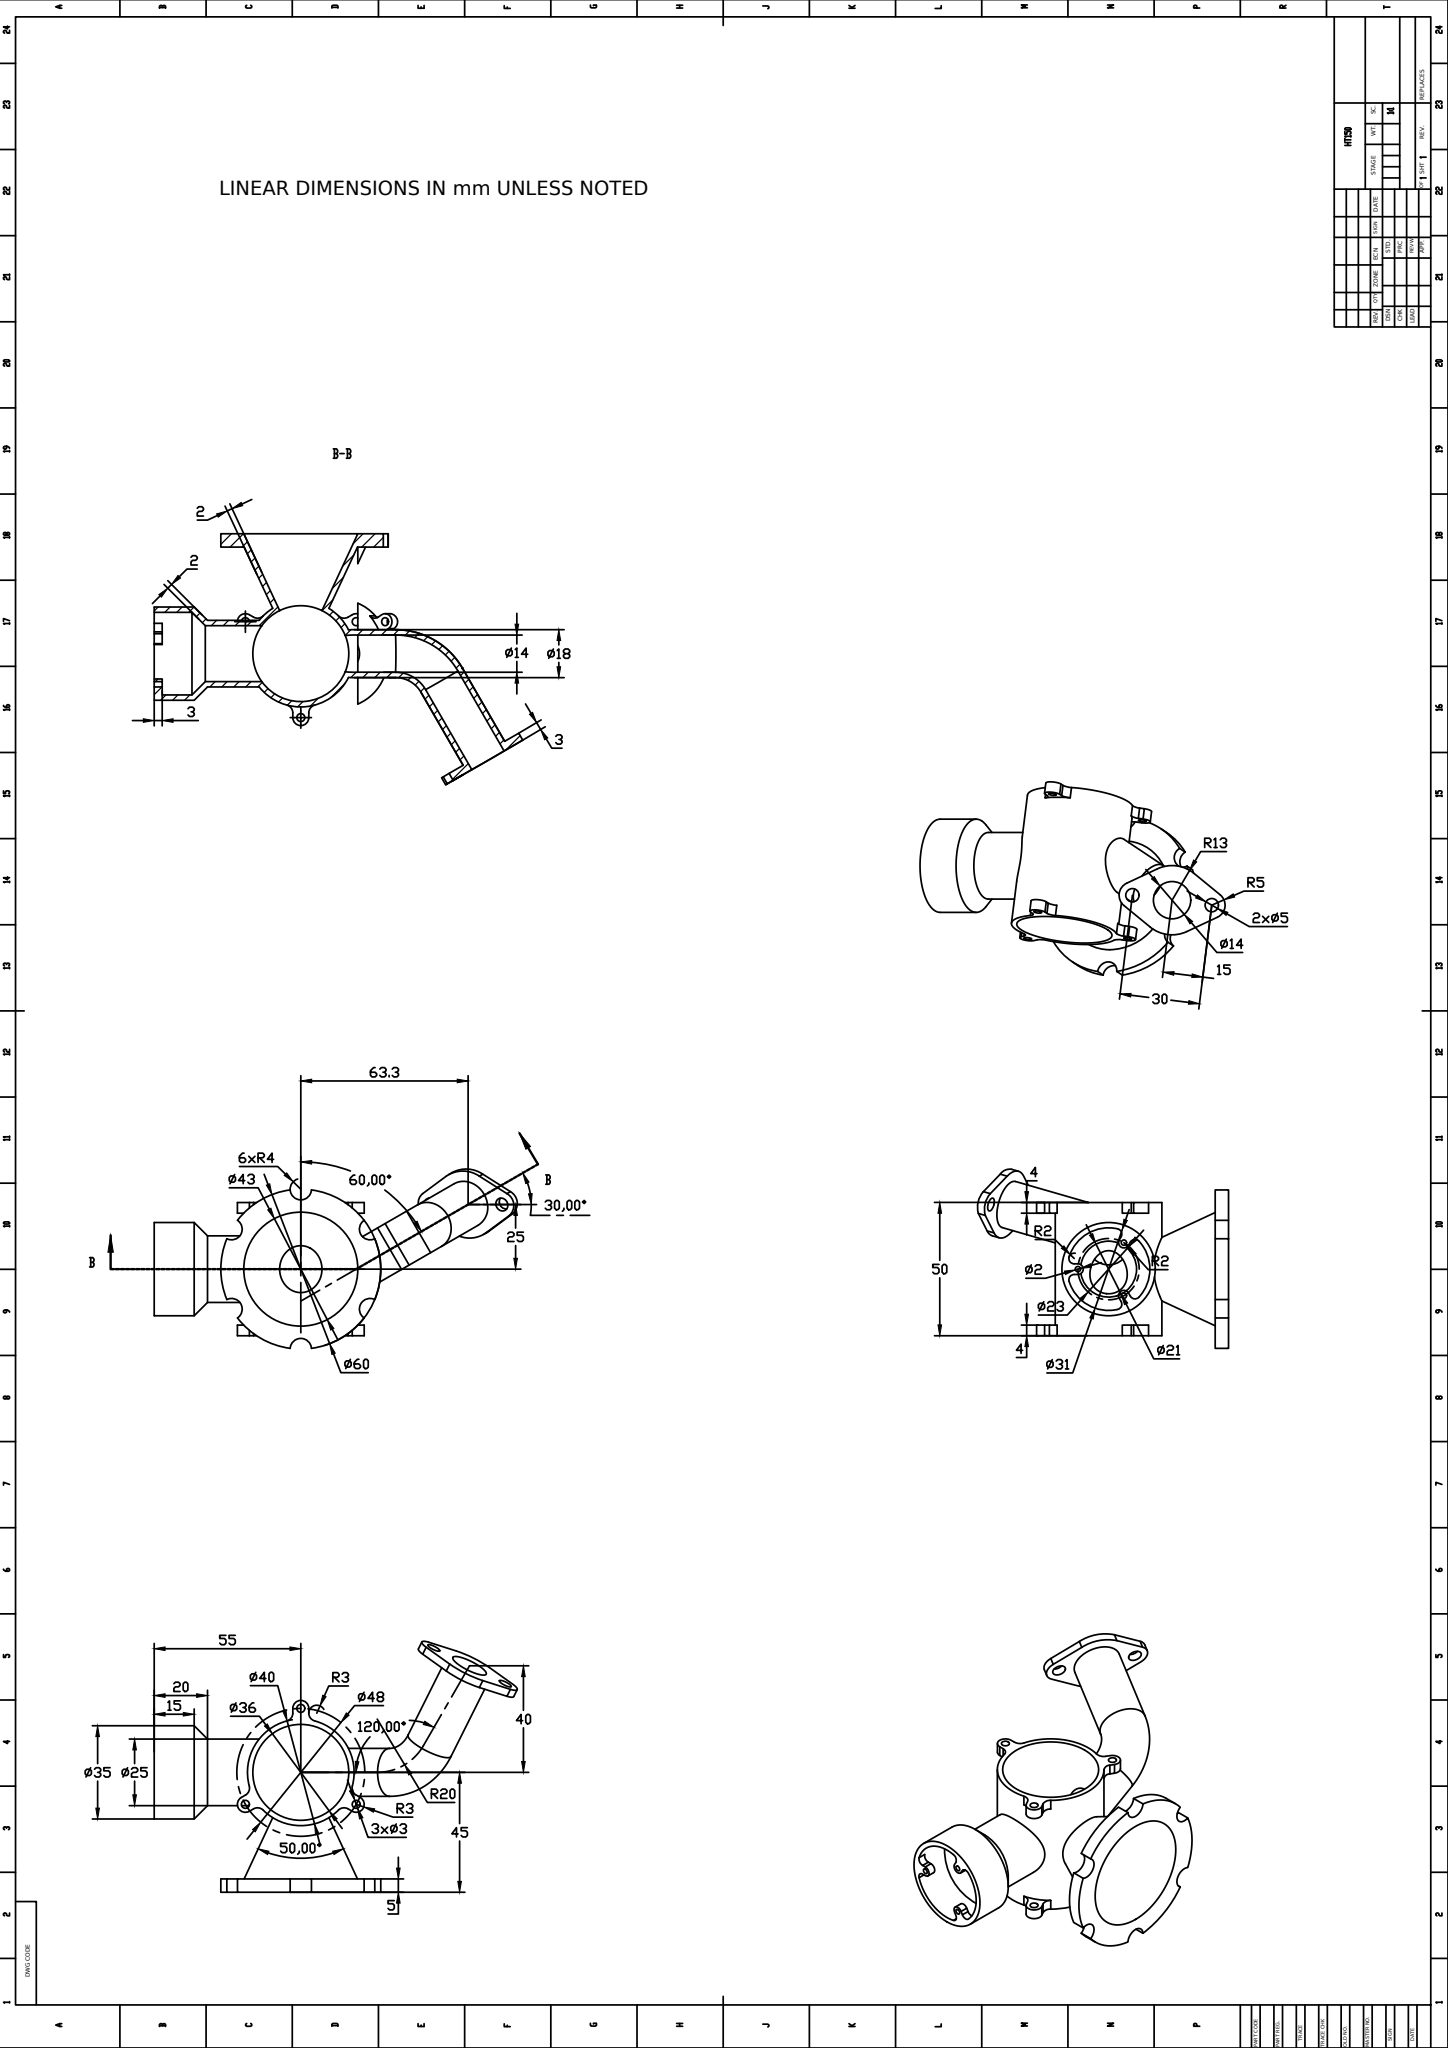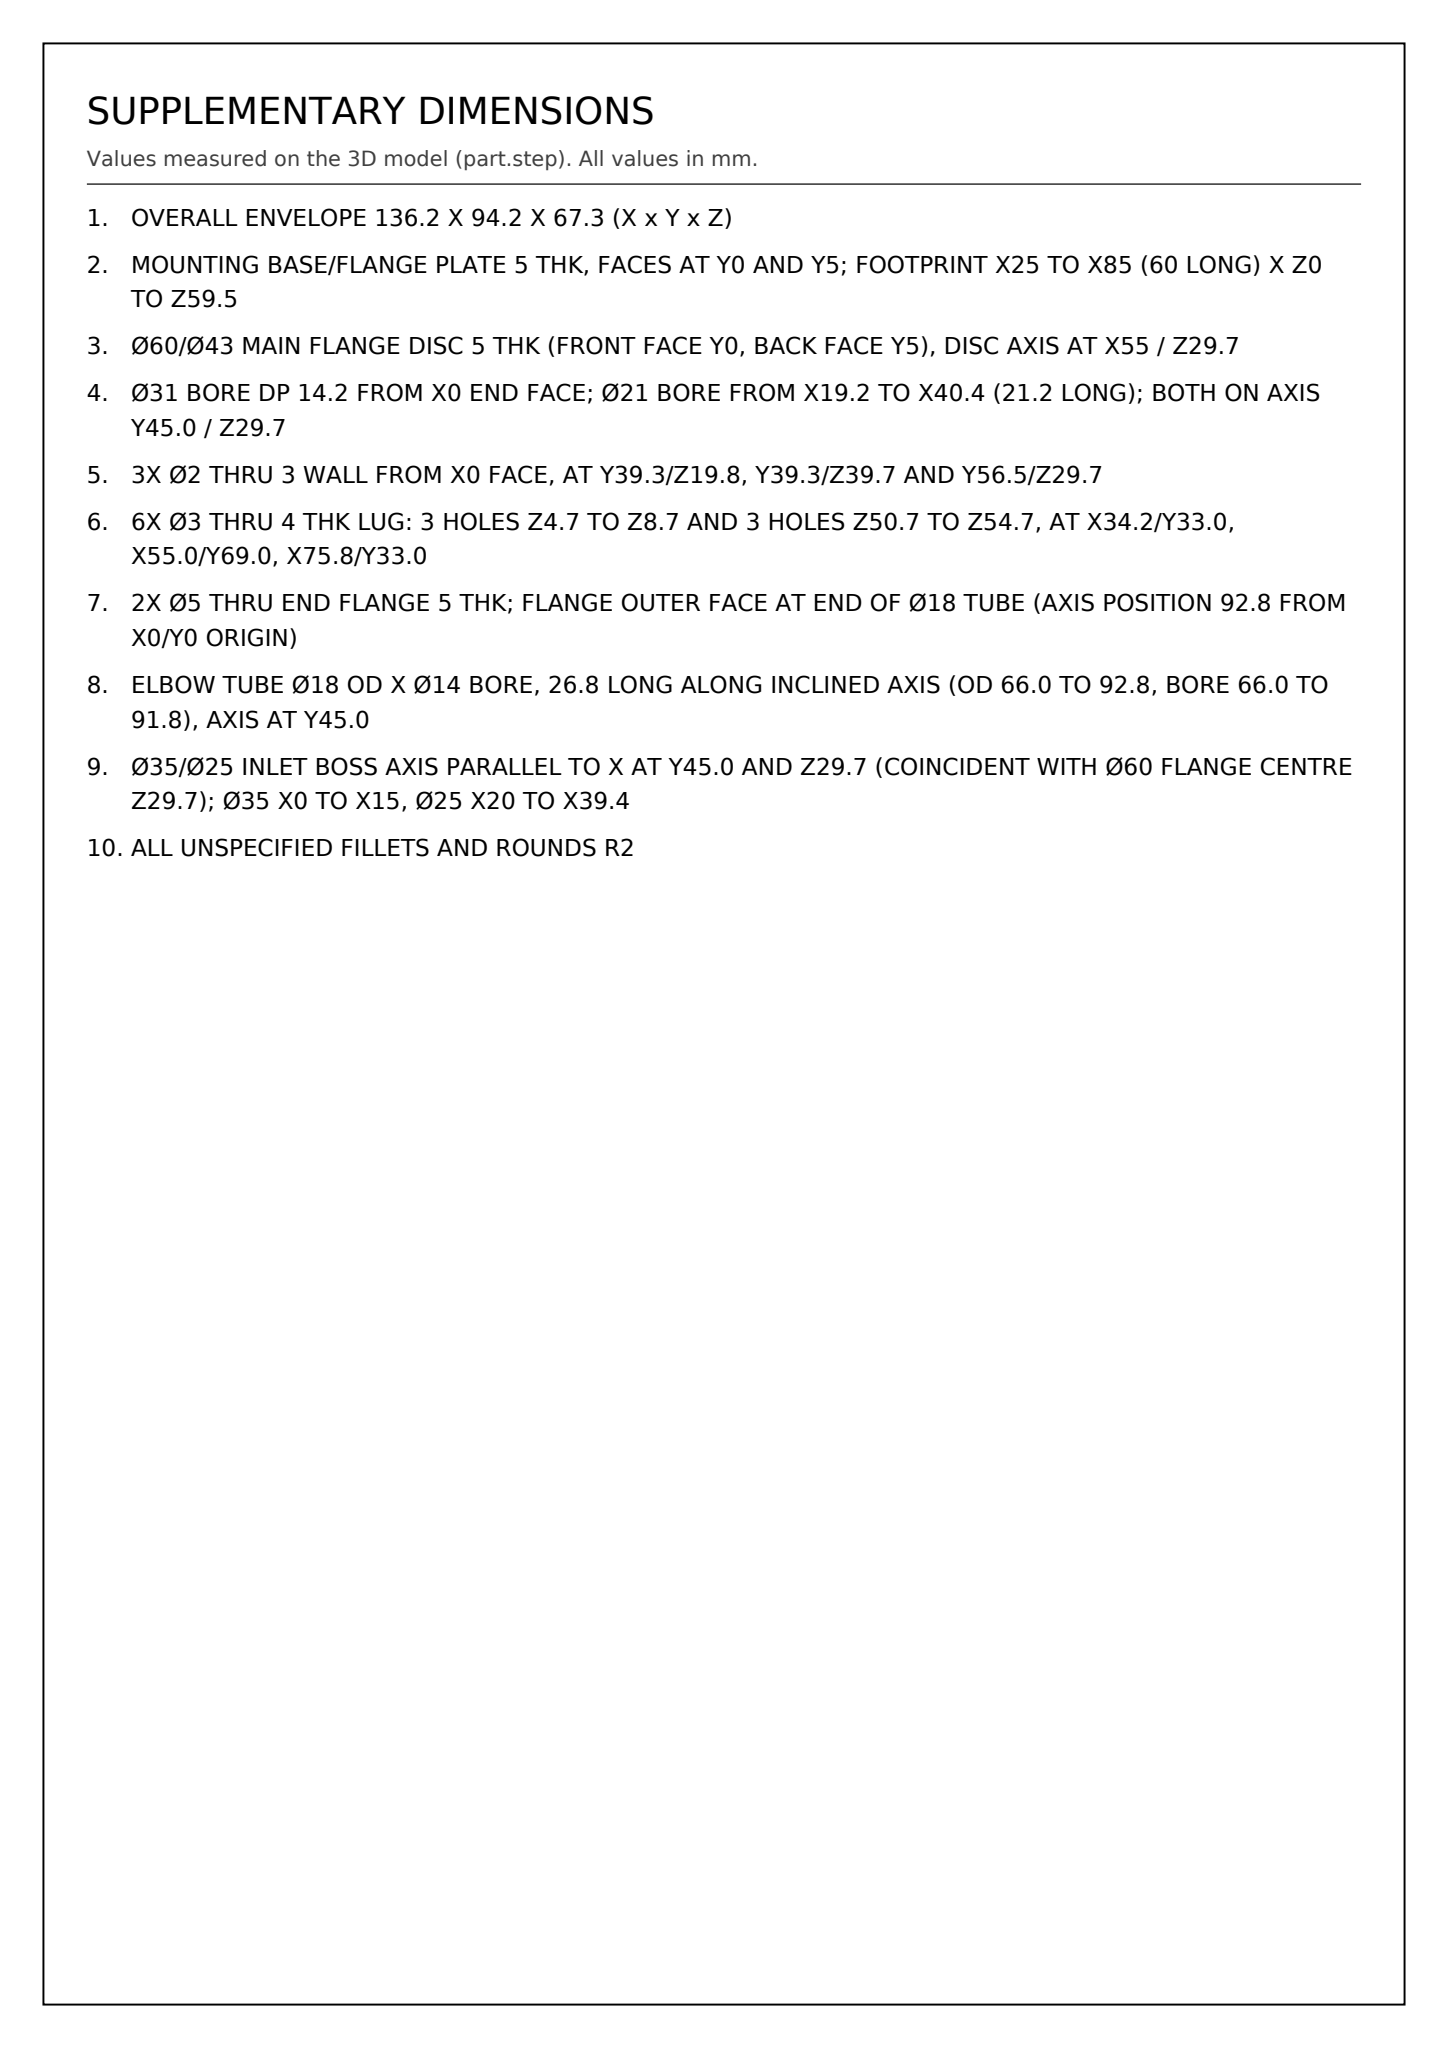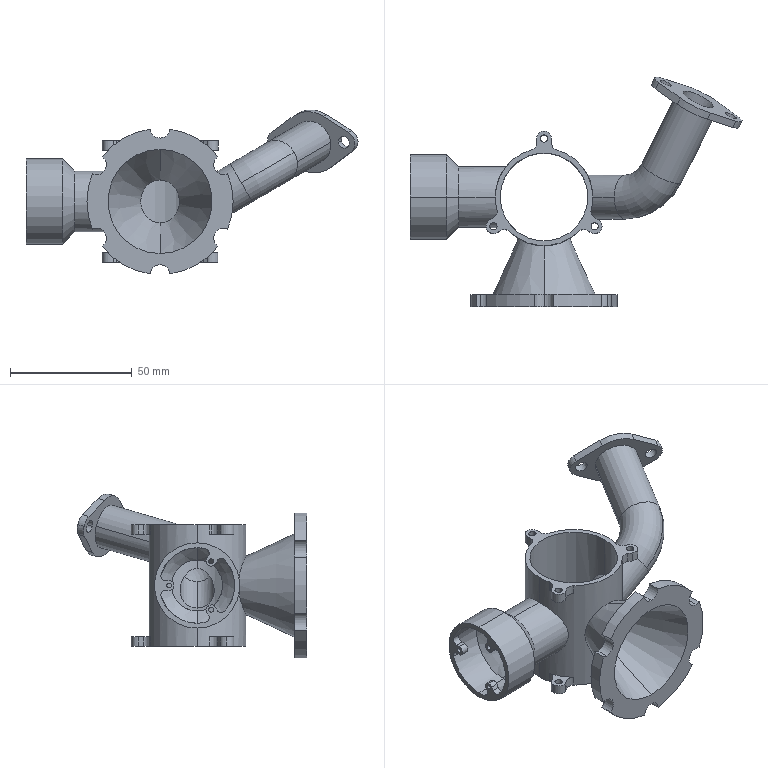Part | SolidWorks | mm | 1 solid | 145 faces | box 136.22 x 94.21 x 67.32 mm | volume 38016 mm3 | cylinder 95 | plane 38 | cone 8 | torus 4 | commonest cylinder face diameters 6 x22 3 x12 4 x11 8 x9 2 x6 60 x6 5 x4 14 x4
Drawing notes:
OVERALL ENVELOPE 136.2 X 94.2 X 67.3 (X x Y x Z) | from the solid: bbox_xyz [136.225, 94.208, 67.321]
MOUNTING BASE/FLANGE PLATE 5 THK, FACES AT Y0 AND Y5; FOOTPRINT X25 TO X85 (60 LONG) X Z0 TO Z59.5 | from the solid: axis_planes normal y at offset 0.0 and 5.0, extent x[25,85] z[0,59.5]
Ø60/Ø43 MAIN FLANGE DISC 5 THK (FRONT FACE Y0, BACK FACE Y5), DISC AXIS AT X55 / Z29.7 | from the solid: convex arc 60.0 axis y at [55.0,null,29.7] from 0.0 to 5.0
Ø31 BORE DP 14.2 FROM X0 END FACE; Ø21 BORE FROM X19.2 TO X40.4 (21.2 LONG); BOTH ON AXIS Y45.0 / Z29.7 | from the solid: hole/bore 31.0 axis x from 0.0 to 14.2 and hole/bore 21.0 axis x from 19.2 to 40.4, axis [null,45.0,29.7]
3X Ø2 THRU 3 WALL FROM X0 FACE, AT Y39.3/Z19.8, Y39.3/Z39.7 AND Y56.5/Z29.7 | from the solid: hole/bore 2.0 axis x from 0.0 to 3.0 at [null,39.3,19.8], [null,39.3,39.7], [null,56.5,29.7]
6X Ø3 THRU 4 THK LUG: 3 HOLES Z4.7 TO Z8.7 AND 3 HOLES Z50.7 TO Z54.7, AT X34.2/Y33.0, X55.0/Y69.0, X75.8/Y33.0 | from the solid: hole/bore 3.0 axis z from 4.7 to 8.7 and 50.7 to 54.7 at [34.2,33.0],[55.0,69.0],[75.8,33.0]
2X Ø5 THRU END FLANGE 5 THK; FLANGE OUTER FACE AT END OF Ø18 TUBE (AXIS POSITION 92.8 FROM X0/Y0 ORIGIN) | from the solid: concave arc 5.0 inclined from 87.9 to 92.8 and from 74.4 to 79.4; boss/shaft 18.0 inclined to 92.8
ELBOW TUBE Ø18 OD X Ø14 BORE, 26.8 LONG ALONG INCLINED AXIS (OD 66.0 TO 92.8, BORE 66.0 TO 91.8), AXIS AT Y45.0 | from the solid: boss/shaft 18.0 inclined [null,45.0,37.4] from 66.0 to 92.8; hole/bore 14.0 inclined from 66.0 to 91.8
Ø35/Ø25 INLET BOSS AXIS PARALLEL TO X AT Y45.0 AND Z29.7 (COINCIDENT WITH Ø60 FLANGE CENTRE Z29.7); Ø35 X0 TO X15, Ø25 X20 TO X39.4 | from the solid: boss/shaft 35.0 axis x [null,45.0,29.7] from 0.0 to 15.0; boss/shaft 25.0 axis x from 20.0 to 39.4; convex arc 60.0 axis y at [55.0,null,29.7]
ALL UNSPECIFIED FILLETS AND ROUNDS R2 | from the solid: smallest blend features in model are dia 4.0 arcs (R2), e.g. convex arc 4.0 axis x at [null,56.5,29.7]